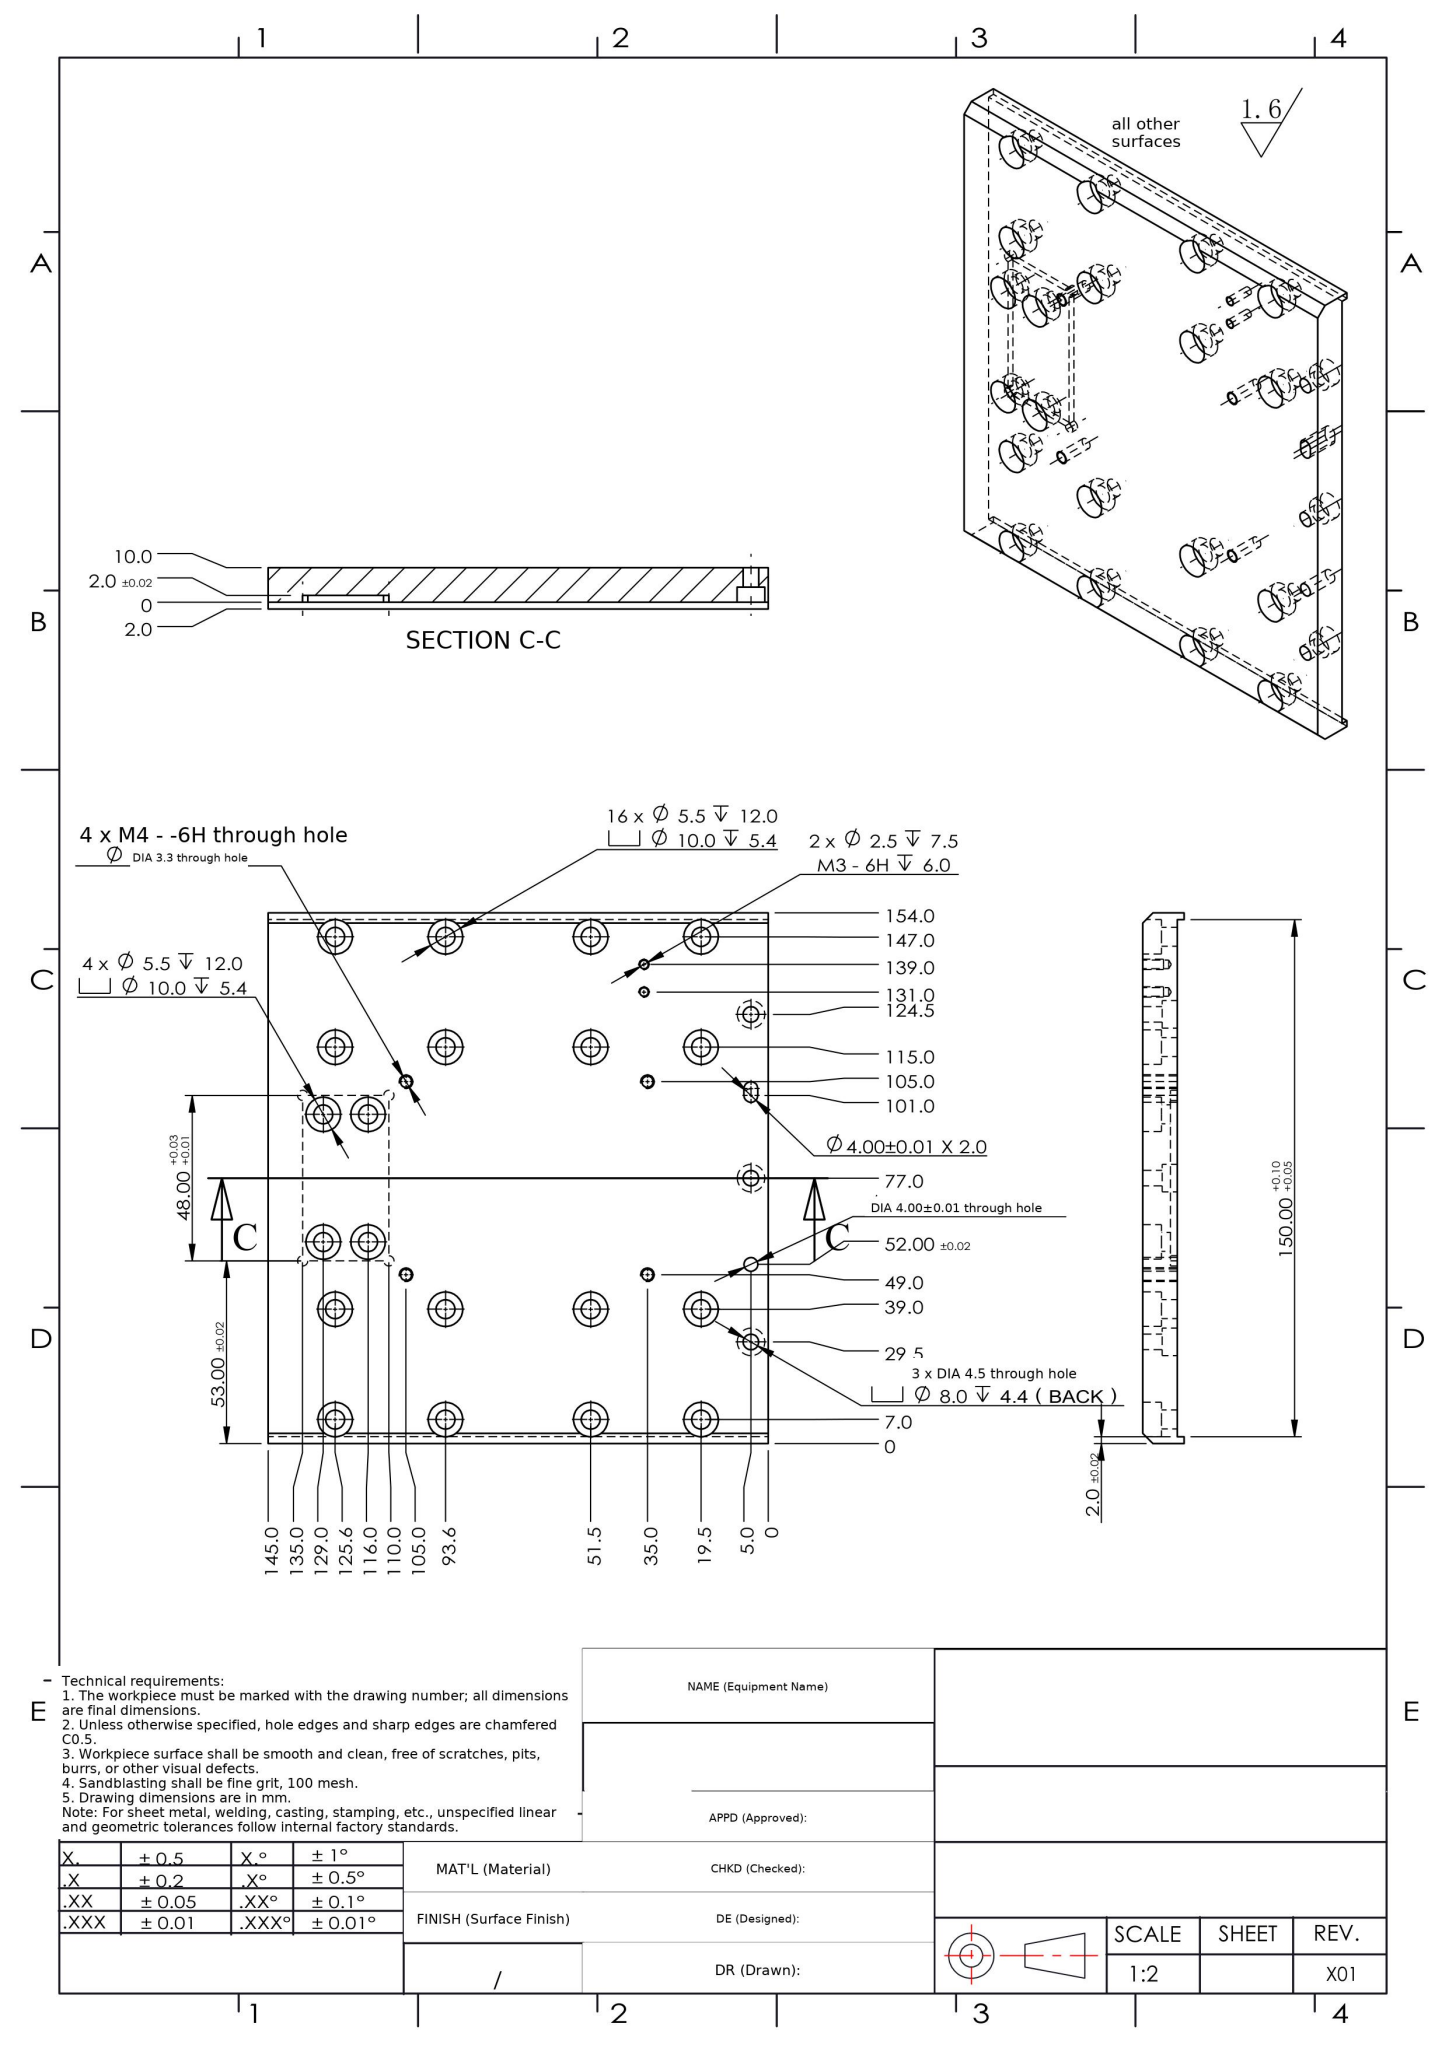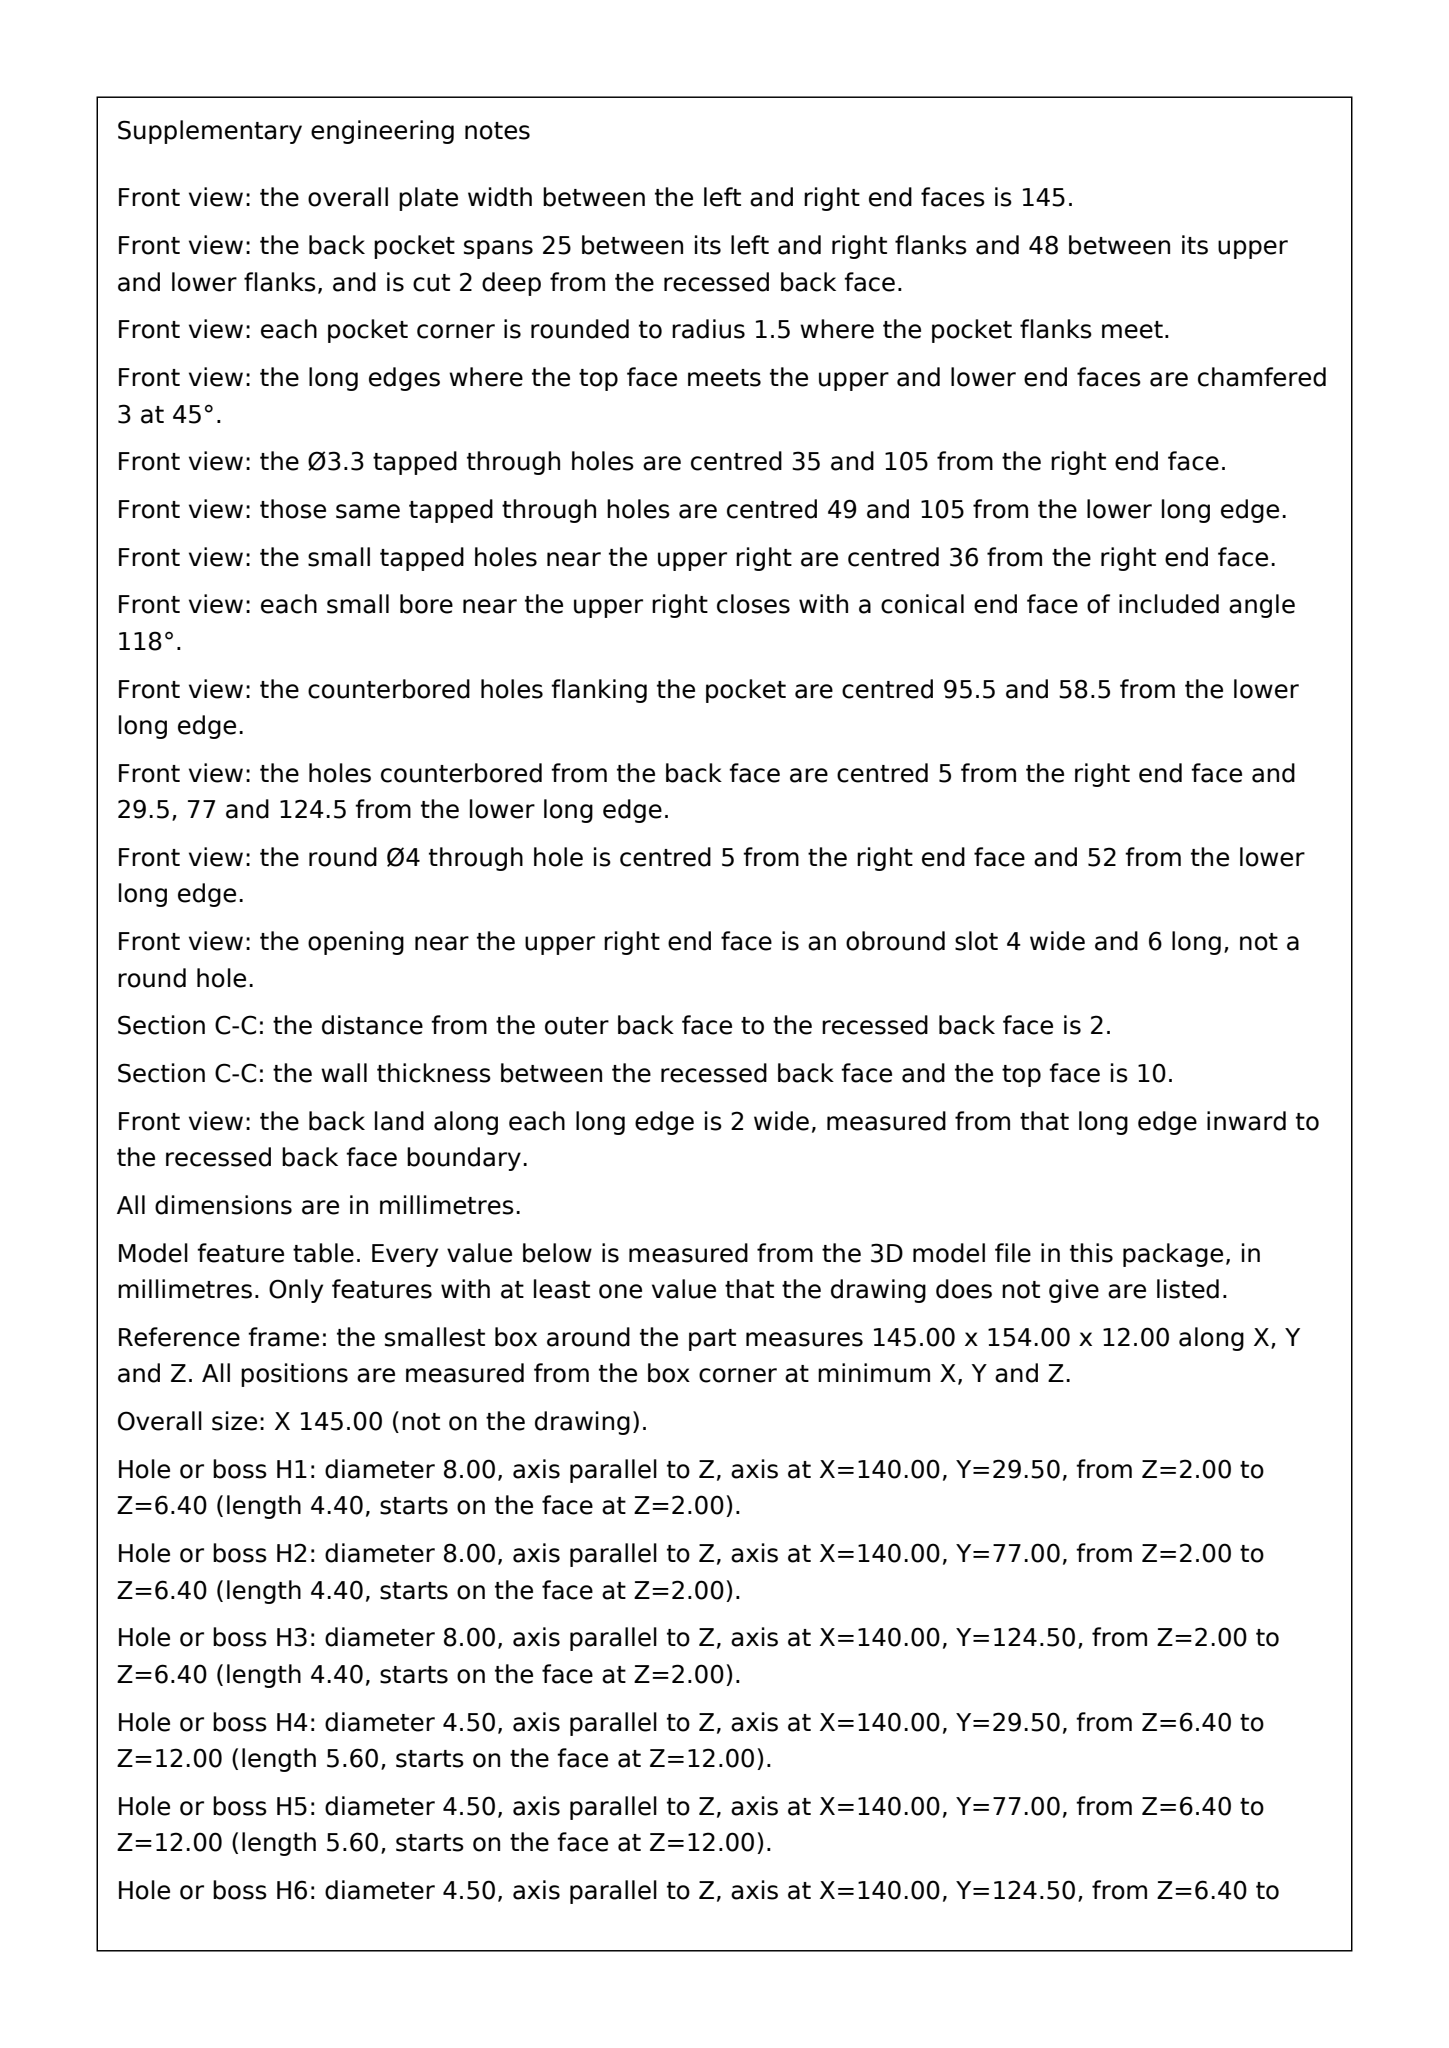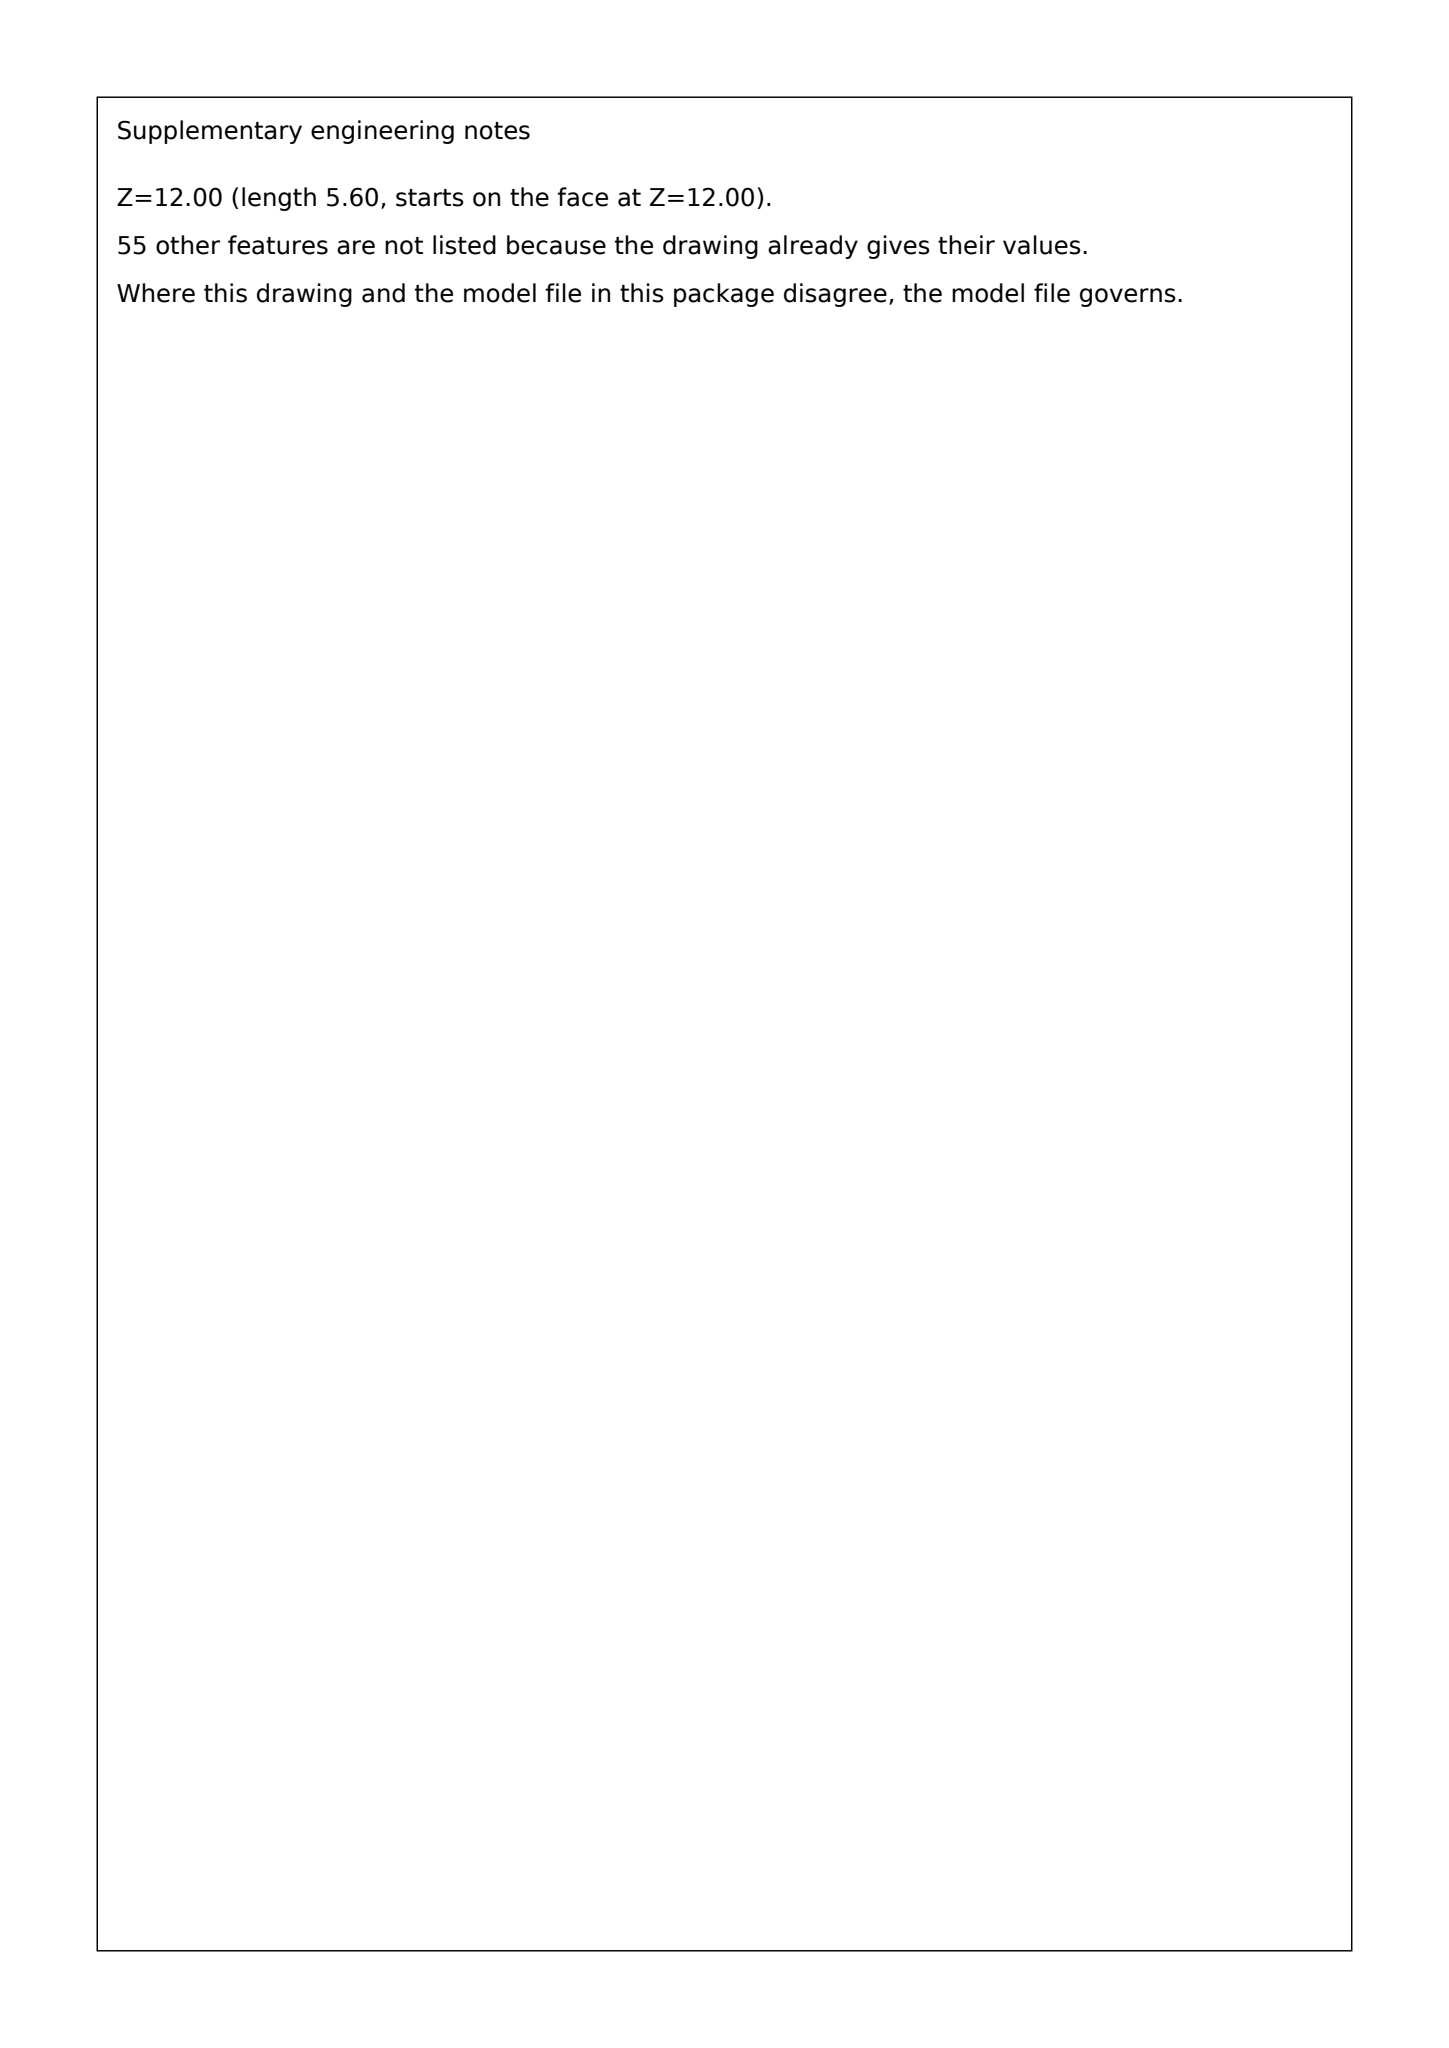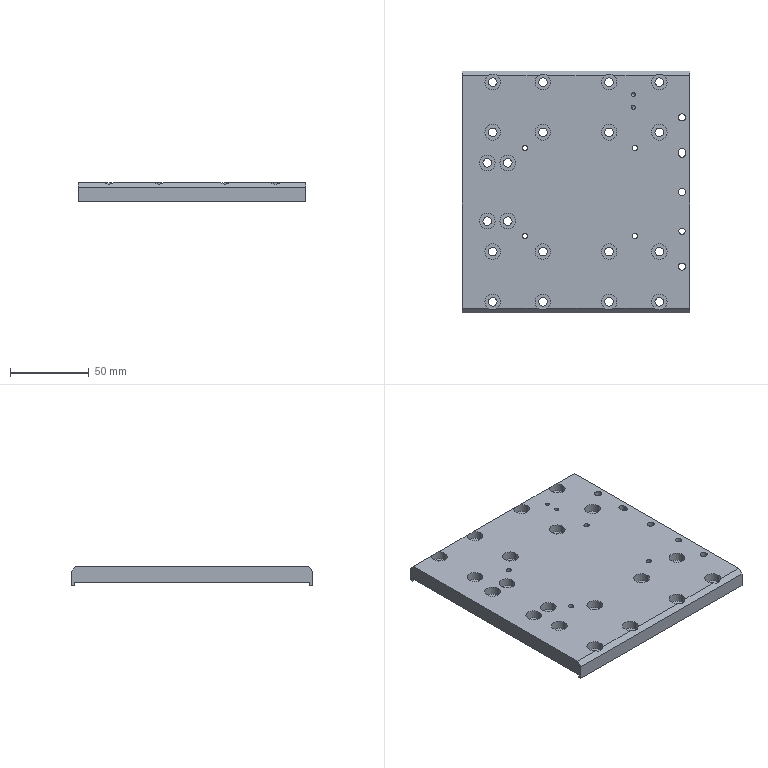Part | SolidWorks | mm | 1 solid | 160 faces | box 145 x 154 x 12 mm | volume 208568 mm3 | cylinder 114 | plane 42 | cone 4 | commonest cylinder face diameters 10 x40 5.5 x40 3.3 x8 3 x6 8 x6 4.5 x6 4 x4 2.5 x4